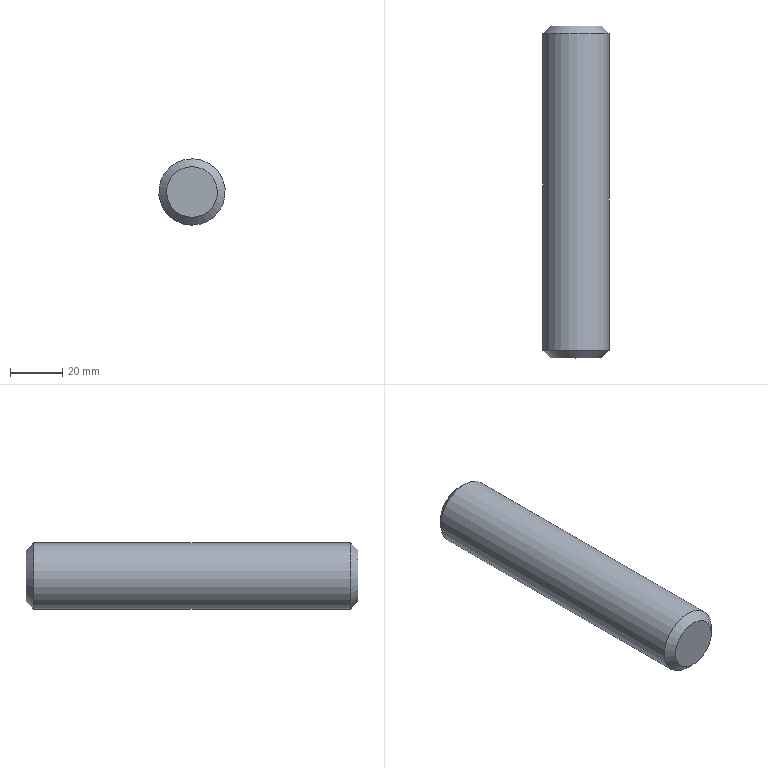Component | NX | PIN_127 | 1 solid | 5 faces | volume 63690 mm3 | plane 2 | cone 2 | cylinder 1 | commonest cylinder face diameters 25.4 x1